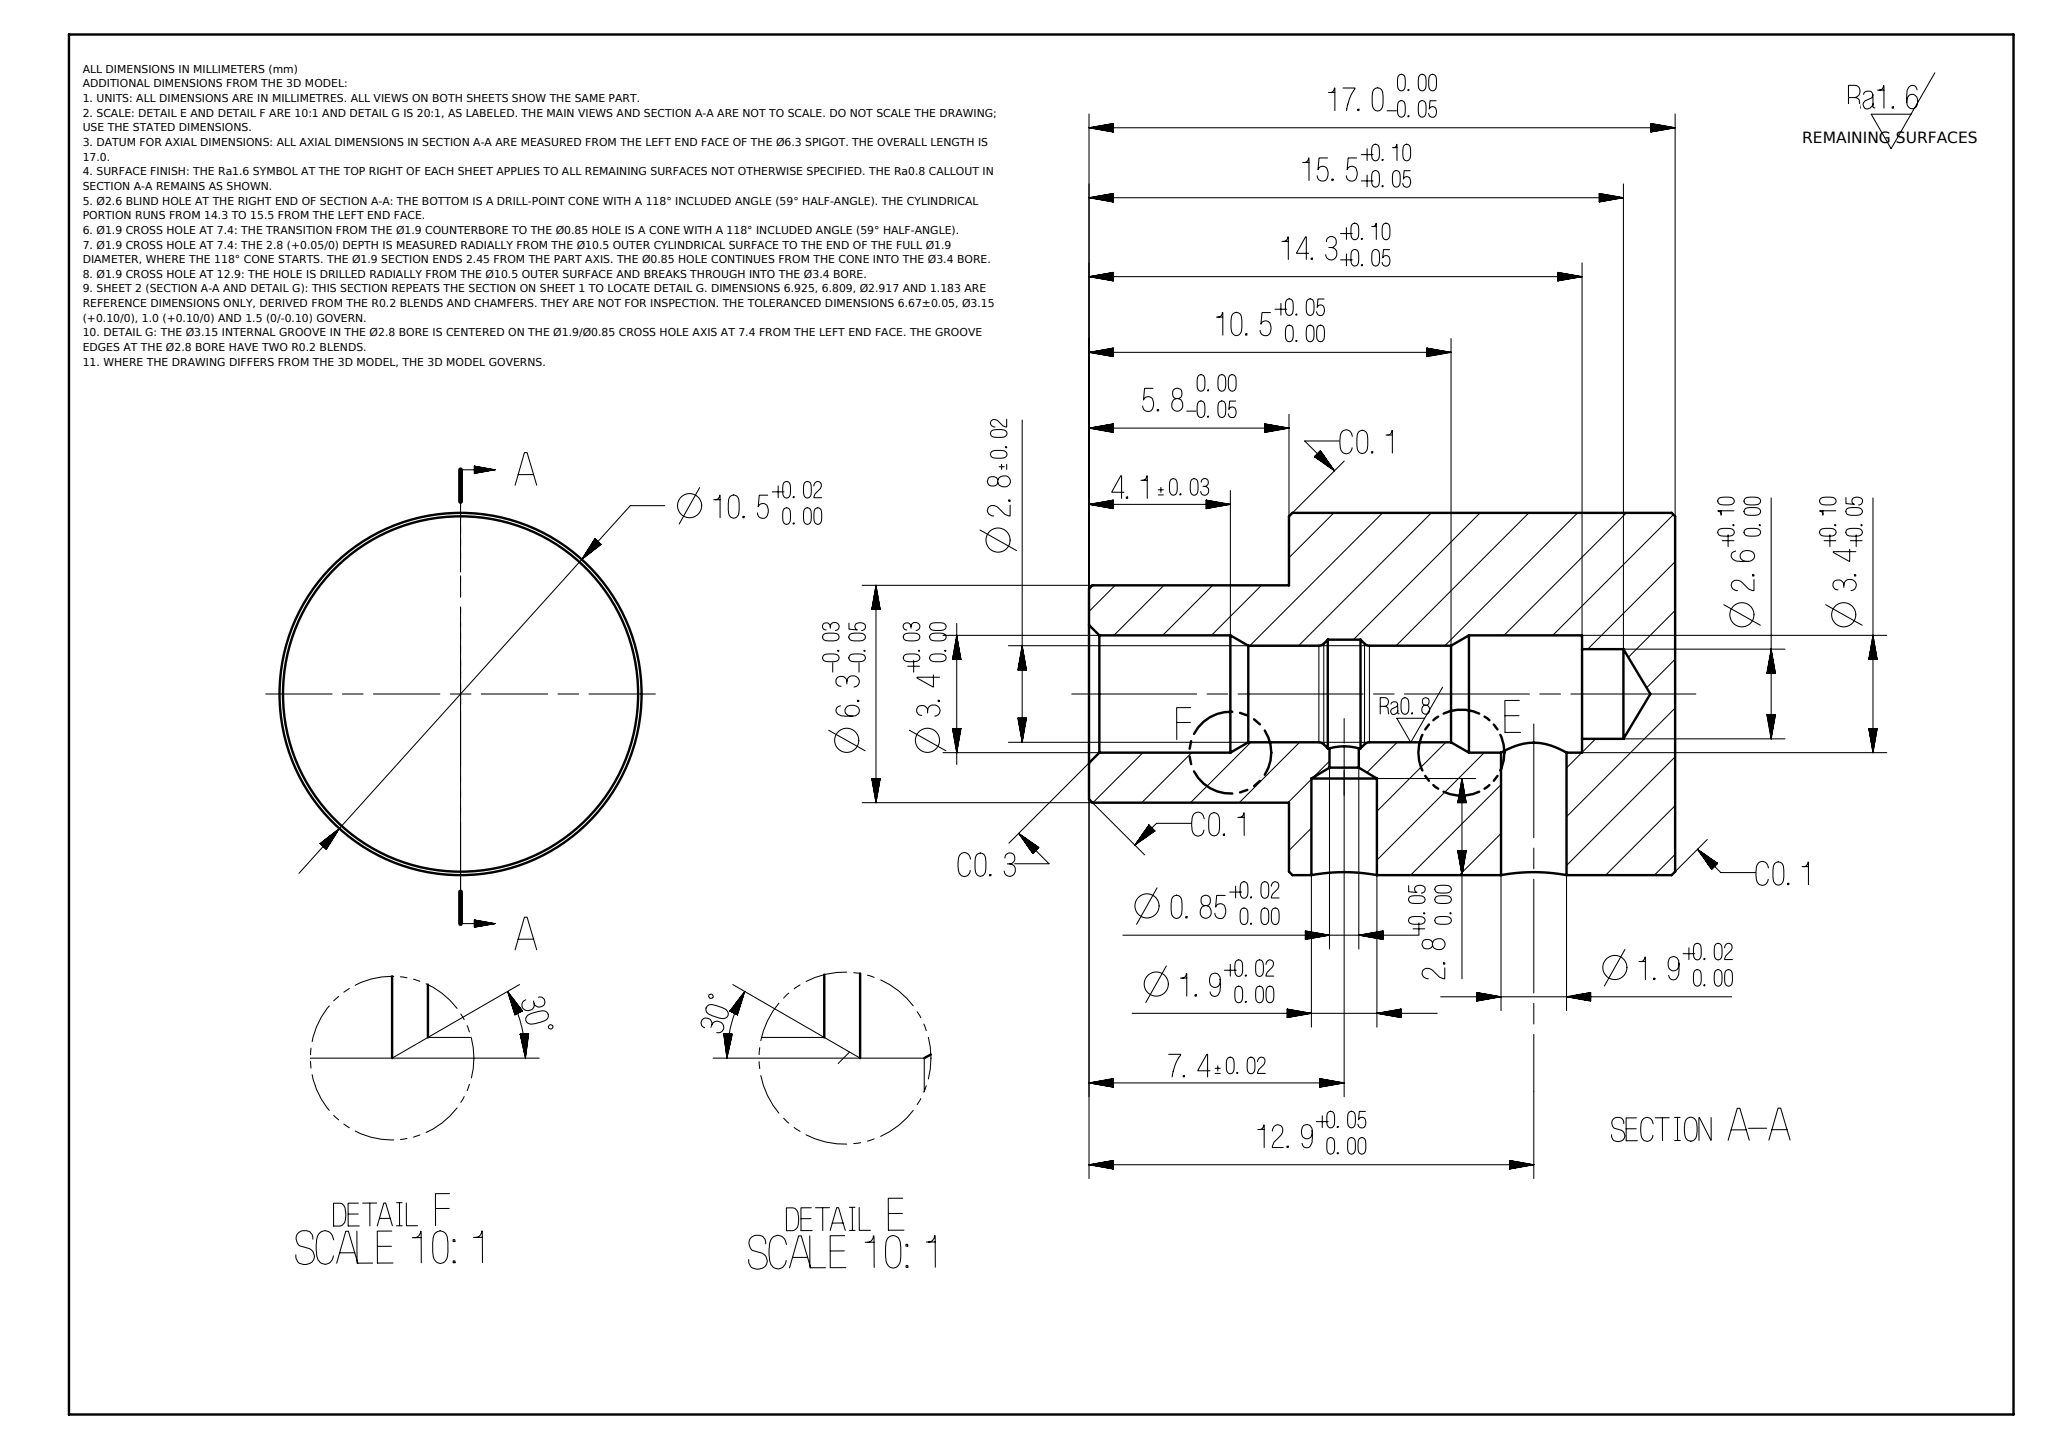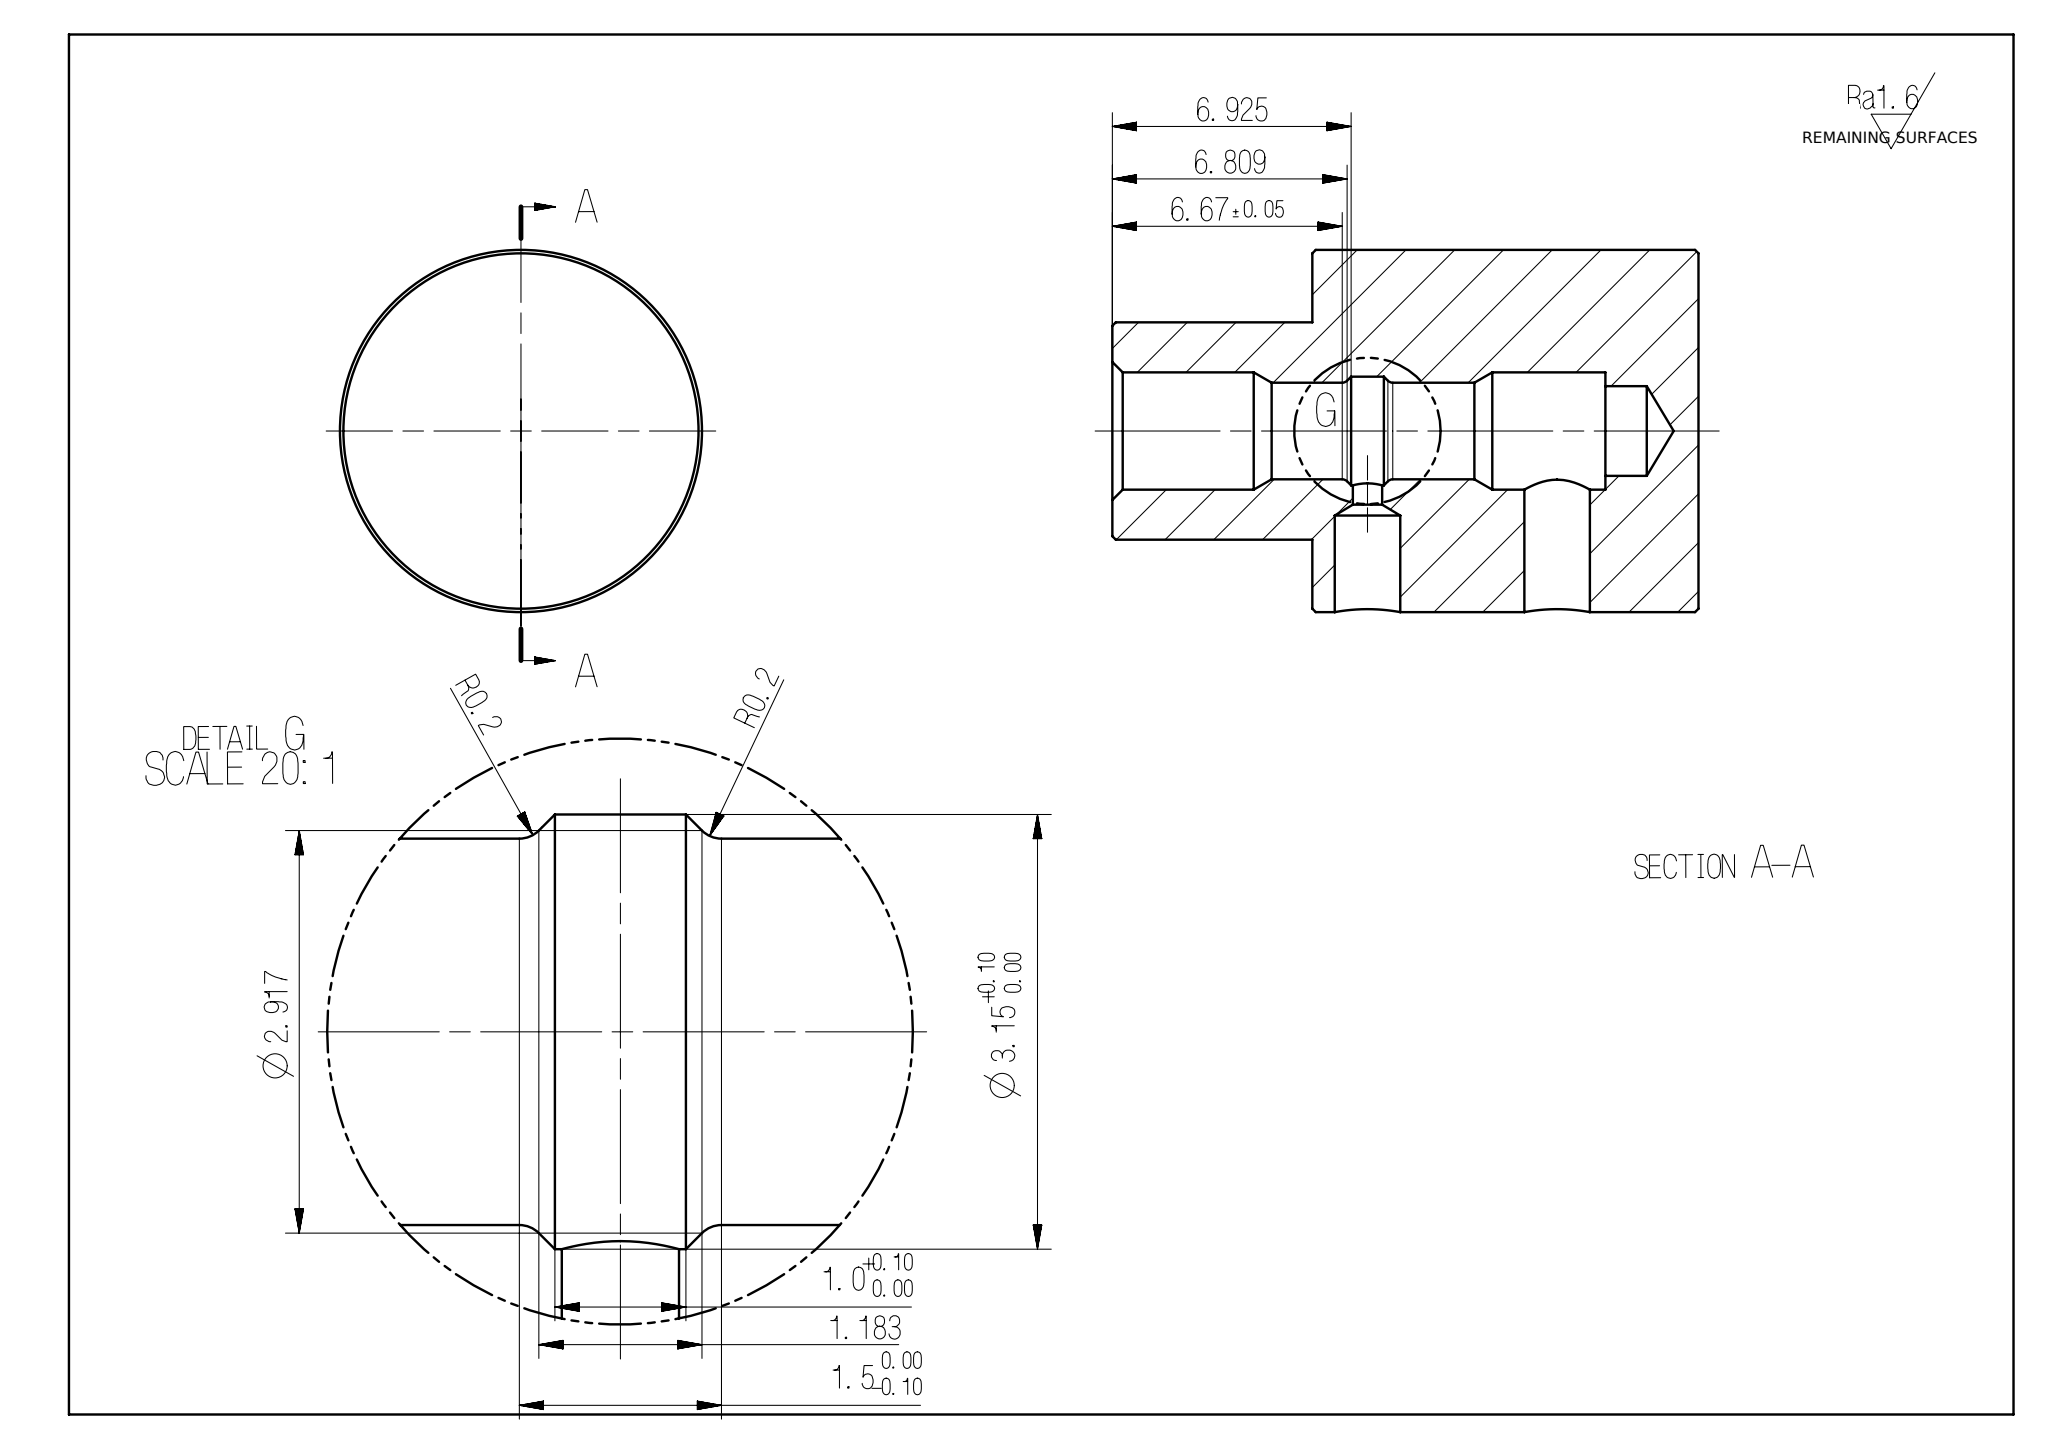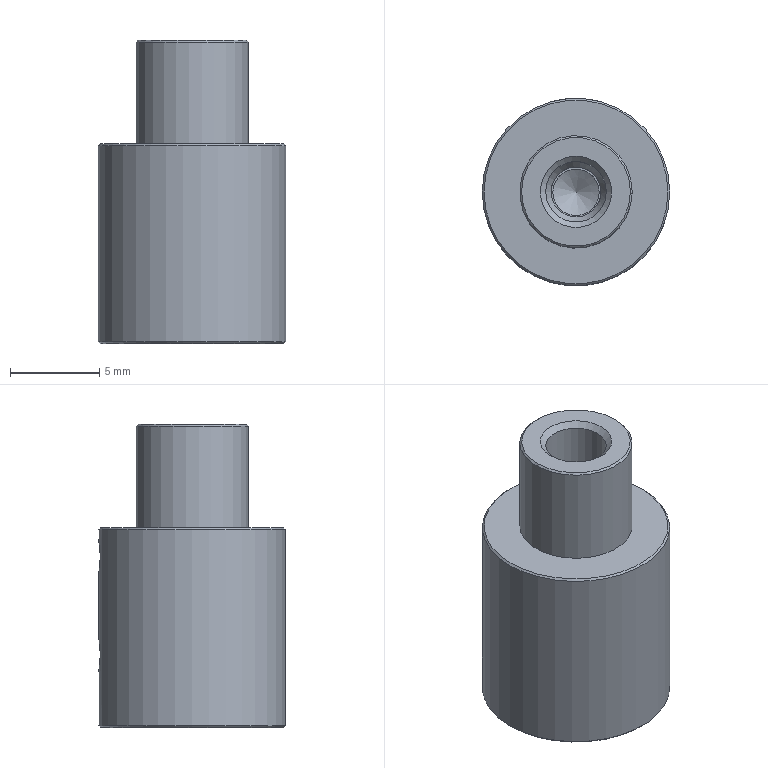Part | NX | mm | 1 solid | 27 faces | box 10.5 x 10.5 x 17 mm | volume 1010 mm3 | cylinder 11 | cone 10 | plane 4 | torus 2 | commonest cylinder face diameters 2.8 x2 3.4 x2 1.9 x2 0.85 x1 10.5 x1 6.3 x1 2.6 x1 3.15 x1
STEP:
#1=CARTESIAN_POINT('',(0.,0.,0.));
#2=DIRECTION('',(0.,0.,1.));
#3=DIRECTION('',(1.,0.,0.));
#4=AXIS2_PLACEMENT_3D('',#1,#2,#3);
#5=(LENGTH_UNIT()NAMED_UNIT(*)SI_UNIT(.MILLI.,.METRE.));
#6=UNCERTAINTY_MEASURE_WITH_UNIT(LENGTH_MEASURE(0.0508),#5,'','');
#7=(NAMED_UNIT(*)PLANE_ANGLE_UNIT()SI_UNIT($,.RADIAN.));
#8=PLANE_ANGLE_MEASURE_WITH_UNIT(PLANE_ANGLE_MEASURE(0.01745),#7);
#9=DIMENSIONAL_EXPONENTS(0.,0.,0.,0.,0.,0.,0.);
#10=(CONVERSION_BASED_UNIT('',#8)NAMED_UNIT(#9)PLANE_ANGLE_UNIT());
#11=(NAMED_UNIT(*)SI_UNIT($,.STERADIAN.)SOLID_ANGLE_UNIT());
#12=(GEOMETRIC_REPRESENTATION_CONTEXT(3)GLOBAL_UNCERTAINTY_ASSIGNED_CONTEXT((#6))GLOBAL_UNIT_ASSIGNED_CONTEXT((#5,#10,#11))REPRESENTATION_CONTEXT('',''));
#13=SHAPE_REPRESENTATION('',(#4),#12);
#14=CARTESIAN_POINT('',(0.,-1.4,10.333));
#15=VERTEX_POINT('',#14);
#16=CARTESIAN_POINT('',(0.,0.,10.333));
#17=DIRECTION('',(0.,-0.,-1.));
#18=DIRECTION('',(0.,-1.,0.));
#19=AXIS2_PLACEMENT_3D('',#16,#17,#18);
#20=CIRCLE('',#19,1.4);
#21=EDGE_CURVE('',#15,#15,#20,.T.);
#22=ORIENTED_EDGE('',*,*,#21,.T.);
#23=EDGE_LOOP('',(#22));
#24=FACE_BOUND('',#23,.T.);
#25=CARTESIAN_POINT('',(-1.4,0.,12.38));
#26=VERTEX_POINT('',#25);
#27=CARTESIAN_POINT('',(0.,0.,12.38));
#28=DIRECTION('',(0.,0.,1.));
#29=DIRECTION('',(-1.,0.,0.));
#30=AXIS2_PLACEMENT_3D('',#27,#28,#29);
#31=CIRCLE('',#30,1.4);
#32=EDGE_CURVE('',#26,#26,#31,.T.);
#33=ORIENTED_EDGE('',*,*,#32,.T.);
#34=EDGE_LOOP('',(#33));
#35=FACE_BOUND('',#34,.T.);
#36=CARTESIAN_POINT('',(0.,0.,6.2));
#37=DIRECTION('',(0.,0.,1.));
#38=DIRECTION('',(1.,0.,0.));
#39=AXIS2_PLACEMENT_3D('',#36,#37,#38);
#40=CYLINDRICAL_SURFACE('',#39,1.4);
#41=ADVANCED_FACE('',(#24,#35),#40,.F.);
#42=CARTESIAN_POINT('',(0.,-1.4,8.867));
#43=VERTEX_POINT('',#42);
#44=CARTESIAN_POINT('',(0.,0.,8.867));
#45=DIRECTION('',(0.,0.,1.));
#46=DIRECTION('',(0.,-1.,0.));
#47=AXIS2_PLACEMENT_3D('',#44,#45,#46);
#48=CIRCLE('',#47,1.4);
#49=EDGE_CURVE('',#43,#43,#48,.T.);
#50=ORIENTED_EDGE('',*,*,#49,.T.);
#51=EDGE_LOOP('',(#50));
#52=FACE_BOUND('',#51,.T.);
#53=CARTESIAN_POINT('',(0.,-1.4,6.5));
#54=VERTEX_POINT('',#53);
#55=CARTESIAN_POINT('',(0.,-0.,6.5));
#56=DIRECTION('',(0.,0.,1.));
#57=DIRECTION('',(0.,-1.,0.));
#58=AXIS2_PLACEMENT_3D('',#55,#56,#57);
#59=CIRCLE('',#58,1.4);
#60=EDGE_CURVE('',#54,#54,#59,.T.);
#61=ORIENTED_EDGE('',*,*,#60,.F.);
#62=EDGE_LOOP('',(#61));
#63=FACE_BOUND('',#62,.T.);
#64=CARTESIAN_POINT('',(0.,0.,6.2));
#65=DIRECTION('',(0.,0.,1.));
#66=DIRECTION('',(1.,0.,0.));
#67=AXIS2_PLACEMENT_3D('',#64,#65,#66);
#68=CYLINDRICAL_SURFACE('',#67,1.4);
#69=ADVANCED_FACE('',(#52,#63),#68,.F.);
#70=CARTESIAN_POINT('',(0.,2.135,10.025));
#71=VERTEX_POINT('',#70);
#72=CARTESIAN_POINT('',(0.,2.135,9.6));
#73=DIRECTION('',(0.,1.,0.));
#74=DIRECTION('',(0.,0.,1.));
#75=AXIS2_PLACEMENT_3D('',#72,#73,#74);
#76=CIRCLE('',#75,0.425);
#77=EDGE_CURVE('',#71,#71,#76,.T.);
#78=ORIENTED_EDGE('',*,*,#77,.T.);
#79=EDGE_LOOP('',(#78));
#80=FACE_BOUND('',#79,.T.);
#81=CARTESIAN_POINT('',(0.425,1.517,9.6));
#82=VERTEX_POINT('',#81);
#83=CARTESIAN_POINT('',(0.425,1.517,9.6));
#84=CARTESIAN_POINT('',(0.425,1.517,9.553));
#85=CARTESIAN_POINT('',(0.4171,1.519,9.506));
#86=CARTESIAN_POINT('',(0.4021,1.523,9.462));
#87=CARTESIAN_POINT('',(0.387,1.527,9.418));
#88=CARTESIAN_POINT('',(0.3645,1.533,9.377));
#89=CARTESIAN_POINT('',(0.3363,1.539,9.34));
#90=CARTESIAN_POINT('',(0.3074,1.545,9.303));
#91=CARTESIAN_POINT('',(0.2718,1.552,9.27));
#92=CARTESIAN_POINT('',(0.2322,1.558,9.244));
#93=CARTESIAN_POINT('',(0.192,1.564,9.218));
#94=CARTESIAN_POINT('',(0.1465,1.569,9.198));
#95=CARTESIAN_POINT('',(0.09951,1.572,9.187));
#96=CARTESIAN_POINT('',(0.05365,1.575,9.176));
#97=CARTESIAN_POINT('',(0.005111,1.576,9.172));
#98=CARTESIAN_POINT('',(-0.0419,1.574,9.177));
#99=CARTESIAN_POINT('',(-0.0877,1.573,9.182));
#100=CARTESIAN_POINT('',(-0.1333,1.57,9.194));
#101=CARTESIAN_POINT('',(-0.175,1.565,9.213));
#102=CARTESIAN_POINT('',(-0.2172,1.561,9.232));
#103=CARTESIAN_POINT('',(-0.2566,1.554,9.258));
#104=CARTESIAN_POINT('',(-0.2903,1.548,9.29));
#105=CARTESIAN_POINT('',(-0.325,1.542,9.322));
#106=CARTESIAN_POINT('',(-0.3546,1.535,9.361));
#107=CARTESIAN_POINT('',(-0.3767,1.529,9.403));
#108=CARTESIAN_POINT('',(-0.3989,1.524,9.446));
#109=CARTESIAN_POINT('',(-0.4141,1.52,9.493));
#110=CARTESIAN_POINT('',(-0.4208,1.518,9.541));
#111=CARTESIAN_POINT('',(-0.4274,1.516,9.587));
#112=CARTESIAN_POINT('',(-0.4261,1.516,9.635));
#113=CARTESIAN_POINT('',(-0.4172,1.519,9.681));
#114=CARTESIAN_POINT('',(-0.4085,1.521,9.726));
#115=CARTESIAN_POINT('',(-0.3922,1.526,9.77));
#116=CARTESIAN_POINT('',(-0.3697,1.531,9.81));
#117=CARTESIAN_POINT('',(-0.3468,1.537,9.85));
#118=CARTESIAN_POINT('',(-0.3167,1.543,9.887));
#119=CARTESIAN_POINT('',(-0.2819,1.55,9.918));
#120=CARTESIAN_POINT('',(-0.2461,1.556,9.95));
#121=CARTESIAN_POINT('',(-0.2043,1.562,9.976));
#122=CARTESIAN_POINT('',(-0.1597,1.567,9.994));
#123=CARTESIAN_POINT('',(-0.1155,1.571,10.012));
#124=CARTESIAN_POINT('',(-0.06734,1.574,10.022));
#125=CARTESIAN_POINT('',(-0.01948,1.575,10.025));
#126=CARTESIAN_POINT('',(0.02689,1.575,10.027));
#127=CARTESIAN_POINT('',(0.07428,1.574,10.021));
#128=CARTESIAN_POINT('',(0.1187,1.571,10.008));
#129=CARTESIAN_POINT('',(0.1629,1.567,9.995));
#130=CARTESIAN_POINT('',(0.2053,1.562,9.975));
#131=CARTESIAN_POINT('',(0.2428,1.556,9.949));
#132=CARTESIAN_POINT('',(0.2814,1.55,9.922));
#133=CARTESIAN_POINT('',(0.3158,1.543,9.888));
#134=CARTESIAN_POINT('',(0.3435,1.537,9.85));
#135=CARTESIAN_POINT('',(0.3717,1.531,9.812));
#136=CARTESIAN_POINT('',(0.3937,1.525,9.767));
#137=CARTESIAN_POINT('',(0.4074,1.521,9.721));
#138=CARTESIAN_POINT('',(0.419,1.518,9.682));
#139=CARTESIAN_POINT('',(0.425,1.517,9.641));
#140=CARTESIAN_POINT('',(0.425,1.517,9.6));
#141=B_SPLINE_CURVE_WITH_KNOTS('',3,(#83,#84,#85,#86,#87,#88,#89,#90,#91,#92,#93,#94,#95,#96,#97,#98,#99,#100,#101,#102,#103,#104,#105,#106,#107,#108,#109,#110,#111,#112,#113,#114,#115,#116,#117,#118,#119,#120,#121,#122,#123,#124,#125,#126,#127,#128,#129,#130,#131,#132,#133,#134,#135,#136,#137,#138,#139,#140),.UNSPECIFIED.,.T.,.F.,(1,3,3,3,3,3,3,3,3,3,3,3,3,3,3,3,3,3,3,3,3,1),(-0.04563,0.,0.05236,0.1046,0.1582,0.2126,0.2657,0.3174,0.3697,0.4236,0.4779,0.5305,0.582,0.6347,0.689,0.7428,0.795,0.8468,0.8999,0.9544,1.,1.052),.UNSPECIFIED.);
#142=EDGE_CURVE('',#82,#82,#141,.T.);
#143=ORIENTED_EDGE('',*,*,#142,.F.);
#144=EDGE_LOOP('',(#143));
#145=FACE_BOUND('',#144,.T.);
#146=CARTESIAN_POINT('',(0.,5.25,9.6));
#147=DIRECTION('',(-0.,-1.,0.));
#148=DIRECTION('',(1.,-0.,0.));
#149=AXIS2_PLACEMENT_3D('',#146,#147,#148);
#150=CYLINDRICAL_SURFACE('',#149,0.425);
#151=ADVANCED_FACE('',(#80,#145),#150,.F.);
#152=CARTESIAN_POINT('',(2.,0.,17.));
#153=VERTEX_POINT('',#152);
#154=CARTESIAN_POINT('',(0.,0.,17.));
#155=DIRECTION('',(0.,0.,-1.));
#156=DIRECTION('',(1.,0.,0.));
#157=AXIS2_PLACEMENT_3D('',#154,#155,#156);
#158=CIRCLE('',#157,2.);
#159=EDGE_CURVE('',#153,#153,#158,.T.);
#160=ORIENTED_EDGE('',*,*,#159,.T.);
#161=EDGE_LOOP('',(#160));
#162=FACE_BOUND('',#161,.T.);
#163=CARTESIAN_POINT('',(3.05,0.,17.));
#164=VERTEX_POINT('',#163);
#165=CARTESIAN_POINT('',(0.,0.,17.));
#166=DIRECTION('',(0.,0.,1.));
#167=DIRECTION('',(1.,0.,0.));
#168=AXIS2_PLACEMENT_3D('',#165,#166,#167);
#169=CIRCLE('',#168,3.05);
#170=EDGE_CURVE('',#164,#164,#169,.T.);
#171=ORIENTED_EDGE('',*,*,#170,.T.);
#172=EDGE_LOOP('',(#171));
#173=FACE_BOUND('',#172,.T.);
#174=CARTESIAN_POINT('',(0.,0.,17.));
#175=DIRECTION('',(0.,0.,1.));
#176=DIRECTION('',(1.,0.,0.));
#177=AXIS2_PLACEMENT_3D('',#174,#175,#176);
#178=PLANE('',#177);
#179=ADVANCED_FACE('',(#162,#173),#178,.T.);
#180=CARTESIAN_POINT('',(-5.15,0.,0.));
#181=VERTEX_POINT('',#180);
#182=CARTESIAN_POINT('',(0.,0.,0.));
#183=DIRECTION('',(0.,0.,-1.));
#184=DIRECTION('',(-1.,0.,0.));
#185=AXIS2_PLACEMENT_3D('',#182,#183,#184);
#186=CIRCLE('',#185,5.15);
#187=EDGE_CURVE('',#181,#181,#186,.T.);
#188=ORIENTED_EDGE('',*,*,#187,.T.);
#189=EDGE_LOOP('',(#188));
#190=FACE_OUTER_BOUND('',#189,.T.);
#191=CARTESIAN_POINT('',(0.,0.,0.));
#192=DIRECTION('',(0.,0.,-1.));
#193=DIRECTION('',(-1.,0.,0.));
#194=AXIS2_PLACEMENT_3D('',#191,#192,#193);
#195=PLANE('',#194);
#196=ADVANCED_FACE('',(#190),#195,.T.);
#197=CARTESIAN_POINT('',(0.,5.25,8.65));
#198=VERTEX_POINT('',#197);
#199=CARTESIAN_POINT('',(0.,5.25,8.65));
#200=CARTESIAN_POINT('',(-0.1054,5.25,8.65));
#201=CARTESIAN_POINT('',(-0.2122,5.247,8.668));
#202=CARTESIAN_POINT('',(-0.3116,5.241,8.703));
#203=CARTESIAN_POINT('',(-0.4109,5.235,8.737));
#204=CARTESIAN_POINT('',(-0.5056,5.226,8.789));
#205=CARTESIAN_POINT('',(-0.588,5.217,8.854));
#206=CARTESIAN_POINT('',(-0.6712,5.208,8.919));
#207=CARTESIAN_POINT('',(-0.7443,5.197,9.));
#208=CARTESIAN_POINT('',(-0.8012,5.189,9.09));
#209=CARTESIAN_POINT('',(-0.8586,5.18,9.18));
#210=CARTESIAN_POINT('',(-0.9012,5.172,9.281));
#211=CARTESIAN_POINT('',(-0.9254,5.168,9.385));
#212=CARTESIAN_POINT('',(-0.9494,5.164,9.488));
#213=CARTESIAN_POINT('',(-0.9559,5.162,9.597));
#214=CARTESIAN_POINT('',(-0.9444,5.164,9.703));
#215=CARTESIAN_POINT('',(-0.9331,5.166,9.807));
#216=CARTESIAN_POINT('',(-0.904,5.172,9.91));
#217=CARTESIAN_POINT('',(-0.8595,5.179,10.005));
#218=CARTESIAN_POINT('',(-0.8148,5.187,10.1));
#219=CARTESIAN_POINT('',(-0.7533,5.196,10.188));
#220=CARTESIAN_POINT('',(-0.6801,5.206,10.263));
#221=CARTESIAN_POINT('',(-0.6058,5.215,10.339));
#222=CARTESIAN_POINT('',(-0.5173,5.225,10.404));
#223=CARTESIAN_POINT('',(-0.4219,5.233,10.451));
#224=CARTESIAN_POINT('',(-0.3263,5.241,10.499));
#225=CARTESIAN_POINT('',(-0.221,5.246,10.53));
#226=CARTESIAN_POINT('',(-0.1149,5.249,10.543));
#227=CARTESIAN_POINT('',(-0.01021,5.251,10.556));
#228=CARTESIAN_POINT('',(0.09817,5.25,10.551));
#229=CARTESIAN_POINT('',(0.2012,5.246,10.528));
#230=CARTESIAN_POINT('',(0.3034,5.242,10.506));
#231=CARTESIAN_POINT('',(0.4032,5.235,10.467));
#232=CARTESIAN_POINT('',(0.4924,5.227,10.412));
#233=CARTESIAN_POINT('',(0.5826,5.218,10.358));
#234=CARTESIAN_POINT('',(0.6646,5.208,10.287));
#235=CARTESIAN_POINT('',(0.7318,5.199,10.206));
#236=CARTESIAN_POINT('',(0.7998,5.189,10.124));
#237=CARTESIAN_POINT('',(0.8546,5.18,10.029));
#238=CARTESIAN_POINT('',(0.8915,5.174,9.928));
#239=CARTESIAN_POINT('',(0.9283,5.167,9.828));
#240=CARTESIAN_POINT('',(0.9483,5.164,9.721));
#241=CARTESIAN_POINT('',(0.9499,5.163,9.614));
#242=CARTESIAN_POINT('',(0.9514,5.163,9.509));
#243=CARTESIAN_POINT('',(0.9351,5.166,9.402));
#244=CARTESIAN_POINT('',(0.9023,5.172,9.303));
#245=CARTESIAN_POINT('',(0.8695,5.178,9.203));
#246=CARTESIAN_POINT('',(0.8195,5.186,9.108));
#247=CARTESIAN_POINT('',(0.7563,5.195,9.025));
#248=CARTESIAN_POINT('',(0.6922,5.205,8.941));
#249=CARTESIAN_POINT('',(0.6128,5.215,8.866));
#250=CARTESIAN_POINT('',(0.5245,5.224,8.808));
#251=CARTESIAN_POINT('',(0.4355,5.233,8.749));
#252=CARTESIAN_POINT('',(0.3348,5.24,8.705));
#253=CARTESIAN_POINT('',(0.231,5.245,8.679));
#254=CARTESIAN_POINT('',(0.1558,5.248,8.66));
#255=CARTESIAN_POINT('',(0.0776,5.25,8.65));
#256=CARTESIAN_POINT('',(0.,5.25,8.65));
#257=B_SPLINE_CURVE_WITH_KNOTS('',3,(#199,#200,#201,#202,#203,#204,#205,#206,#207,#208,#209,#210,#211,#212,#213,#214,#215,#216,#217,#218,#219,#220,#221,#222,#223,#224,#225,#226,#227,#228,#229,#230,#231,#232,#233,#234,#235,#236,#237,#238,#239,#240,#241,#242,#243,#244,#245,#246,#247,#248,#249,#250,#251,#252,#253,#254,#255,#256),.UNSPECIFIED.,.T.,.F.,(1,3,3,3,3,3,3,3,3,3,3,3,3,3,3,3,3,3,3,3,3,1),(-0.03885,0.,0.05311,0.1062,0.1598,0.2138,0.2673,0.32,0.3731,0.4269,0.4808,0.534,0.5868,0.6401,0.6941,0.7478,0.8007,0.8535,0.9071,0.9611,1.,1.053),.UNSPECIFIED.);
#258=EDGE_CURVE('',#198,#198,#257,.T.);
#259=ORIENTED_EDGE('',*,*,#258,.F.);
#260=EDGE_LOOP('',(#259));
#261=FACE_BOUND('',#260,.T.);
#262=CARTESIAN_POINT('',(-5.25,0.,0.1));
#263=VERTEX_POINT('',#262);
#264=CARTESIAN_POINT('',(0.,0.,0.1));
#265=DIRECTION('',(0.,0.,1.));
#266=DIRECTION('',(-1.,0.,0.));
#267=AXIS2_PLACEMENT_3D('',#264,#265,#266);
#268=CIRCLE('',#267,5.25);
#269=EDGE_CURVE('',#263,#263,#268,.T.);
#270=ORIENTED_EDGE('',*,*,#269,.T.);
#271=EDGE_LOOP('',(#270));
#272=FACE_BOUND('',#271,.T.);
#273=CARTESIAN_POINT('',(5.25,0.,11.1));
#274=VERTEX_POINT('',#273);
#275=CARTESIAN_POINT('',(0.,0.,11.1));
#276=DIRECTION('',(0.,0.,-1.));
#277=DIRECTION('',(1.,0.,0.));
#278=AXIS2_PLACEMENT_3D('',#275,#276,#277);
#279=CIRCLE('',#278,5.25);
#280=EDGE_CURVE('',#274,#274,#279,.T.);
#281=ORIENTED_EDGE('',*,*,#280,.T.);
#282=EDGE_LOOP('',(#281));
#283=FACE_BOUND('',#282,.T.);
#284=CARTESIAN_POINT('',(0.,5.25,5.05));
#285=VERTEX_POINT('',#284);
#286=CARTESIAN_POINT('',(0.,5.25,5.05));
#287=CARTESIAN_POINT('',(0.1054,5.25,5.05));
#288=CARTESIAN_POINT('',(0.2122,5.247,5.032));
#289=CARTESIAN_POINT('',(0.3116,5.241,4.997));
#290=CARTESIAN_POINT('',(0.4109,5.235,4.963));
#291=CARTESIAN_POINT('',(0.5056,5.226,4.911));
#292=CARTESIAN_POINT('',(0.588,5.217,4.846));
#293=CARTESIAN_POINT('',(0.6712,5.208,4.781));
#294=CARTESIAN_POINT('',(0.7443,5.197,4.7));
#295=CARTESIAN_POINT('',(0.8012,5.189,4.61));
#296=CARTESIAN_POINT('',(0.8586,5.18,4.52));
#297=CARTESIAN_POINT('',(0.9012,5.172,4.419));
#298=CARTESIAN_POINT('',(0.9254,5.168,4.315));
#299=CARTESIAN_POINT('',(0.9494,5.164,4.212));
#300=CARTESIAN_POINT('',(0.9559,5.162,4.103));
#301=CARTESIAN_POINT('',(0.9444,5.164,3.997));
#302=CARTESIAN_POINT('',(0.9331,5.166,3.893));
#303=CARTESIAN_POINT('',(0.904,5.172,3.79));
#304=CARTESIAN_POINT('',(0.8595,5.179,3.695));
#305=CARTESIAN_POINT('',(0.8148,5.187,3.6));
#306=CARTESIAN_POINT('',(0.7533,5.196,3.512));
#307=CARTESIAN_POINT('',(0.6801,5.206,3.437));
#308=CARTESIAN_POINT('',(0.6058,5.215,3.361));
#309=CARTESIAN_POINT('',(0.5173,5.225,3.296));
#310=CARTESIAN_POINT('',(0.4219,5.233,3.249));
#311=CARTESIAN_POINT('',(0.3263,5.241,3.201));
#312=CARTESIAN_POINT('',(0.221,5.246,3.17));
#313=CARTESIAN_POINT('',(0.1149,5.249,3.157));
#314=CARTESIAN_POINT('',(0.01021,5.251,3.144));
#315=CARTESIAN_POINT('',(-0.09817,5.25,3.149));
#316=CARTESIAN_POINT('',(-0.2012,5.246,3.172));
#317=CARTESIAN_POINT('',(-0.3034,5.242,3.194));
#318=CARTESIAN_POINT('',(-0.4032,5.235,3.233));
#319=CARTESIAN_POINT('',(-0.4924,5.227,3.288));
#320=CARTESIAN_POINT('',(-0.5826,5.218,3.342));
#321=CARTESIAN_POINT('',(-0.6646,5.208,3.413));
#322=CARTESIAN_POINT('',(-0.7318,5.199,3.494));
#323=CARTESIAN_POINT('',(-0.7998,5.189,3.576));
#324=CARTESIAN_POINT('',(-0.8546,5.18,3.671));
#325=CARTESIAN_POINT('',(-0.8915,5.174,3.772));
#326=CARTESIAN_POINT('',(-0.9283,5.167,3.872));
#327=CARTESIAN_POINT('',(-0.9483,5.164,3.979));
#328=CARTESIAN_POINT('',(-0.9499,5.163,4.086));
#329=CARTESIAN_POINT('',(-0.9514,5.163,4.191));
#330=CARTESIAN_POINT('',(-0.9351,5.166,4.298));
#331=CARTESIAN_POINT('',(-0.9023,5.172,4.397));
#332=CARTESIAN_POINT('',(-0.8695,5.178,4.497));
#333=CARTESIAN_POINT('',(-0.8195,5.186,4.592));
#334=CARTESIAN_POINT('',(-0.7563,5.195,4.675));
#335=CARTESIAN_POINT('',(-0.6922,5.205,4.759));
#336=CARTESIAN_POINT('',(-0.6128,5.215,4.834));
#337=CARTESIAN_POINT('',(-0.5245,5.224,4.892));
#338=CARTESIAN_POINT('',(-0.4355,5.233,4.951));
#339=CARTESIAN_POINT('',(-0.3348,5.24,4.995));
#340=CARTESIAN_POINT('',(-0.231,5.245,5.021));
#341=CARTESIAN_POINT('',(-0.1558,5.248,5.04));
#342=CARTESIAN_POINT('',(-0.0776,5.25,5.05));
#343=CARTESIAN_POINT('',(0.,5.25,5.05));
#344=B_SPLINE_CURVE_WITH_KNOTS('',3,(#286,#287,#288,#289,#290,#291,#292,#293,#294,#295,#296,#297,#298,#299,#300,#301,#302,#303,#304,#305,#306,#307,#308,#309,#310,#311,#312,#313,#314,#315,#316,#317,#318,#319,#320,#321,#322,#323,#324,#325,#326,#327,#328,#329,#330,#331,#332,#333,#334,#335,#336,#337,#338,#339,#340,#341,#342,#343),.UNSPECIFIED.,.T.,.F.,(1,3,3,3,3,3,3,3,3,3,3,3,3,3,3,3,3,3,3,3,3,1),(-0.03885,0.,0.05311,0.1062,0.1598,0.2138,0.2673,0.32,0.3731,0.4269,0.4808,0.534,0.5868,0.6401,0.6941,0.7478,0.8007,0.8535,0.9071,0.9611,1.,1.053),.UNSPECIFIED.);
#345=EDGE_CURVE('',#285,#285,#344,.T.);
#346=ORIENTED_EDGE('',*,*,#345,.F.);
#347=EDGE_LOOP('',(#346));
#348=FACE_BOUND('',#347,.T.);
#349=CARTESIAN_POINT('',(0.,0.,0.));
#350=DIRECTION('',(0.,0.,1.));
#351=DIRECTION('',(1.,0.,0.));
#352=AXIS2_PLACEMENT_3D('',#349,#350,#351);
#353=CYLINDRICAL_SURFACE('',#352,5.25);
#354=ADVANCED_FACE('',(#261,#272,#283,#348),#353,.T.);
#355=CARTESIAN_POINT('',(5.15,0.,11.2));
#356=VERTEX_POINT('',#355);
#357=CARTESIAN_POINT('',(0.,0.,11.2));
#358=DIRECTION('',(0.,0.,1.));
#359=DIRECTION('',(1.,0.,0.));
#360=AXIS2_PLACEMENT_3D('',#357,#358,#359);
#361=CIRCLE('',#360,5.15);
#362=EDGE_CURVE('',#356,#356,#361,.T.);
#363=ORIENTED_EDGE('',*,*,#362,.T.);
#364=EDGE_LOOP('',(#363));
#365=FACE_BOUND('',#364,.T.);
#366=CARTESIAN_POINT('',(3.15,0.,11.2));
#367=VERTEX_POINT('',#366);
#368=CARTESIAN_POINT('',(0.,0.,11.2));
#369=DIRECTION('',(0.,0.,1.));
#370=DIRECTION('',(1.,0.,0.));
#371=AXIS2_PLACEMENT_3D('',#368,#369,#370);
#372=CIRCLE('',#371,3.15);
#373=EDGE_CURVE('',#367,#367,#372,.T.);
#374=ORIENTED_EDGE('',*,*,#373,.F.);
#375=EDGE_LOOP('',(#374));
#376=FACE_BOUND('',#375,.T.);
#377=CARTESIAN_POINT('',(0.,0.,11.2));
#378=DIRECTION('',(0.,0.,1.));
#379=DIRECTION('',(1.,0.,0.));
#380=AXIS2_PLACEMENT_3D('',#377,#378,#379);
#381=PLANE('',#380);
#382=ADVANCED_FACE('',(#365,#376),#381,.T.);
#383=CARTESIAN_POINT('',(3.15,0.,16.9));
#384=VERTEX_POINT('',#383);
#385=CARTESIAN_POINT('',(0.,0.,16.9));
#386=DIRECTION('',(0.,0.,-1.));
#387=DIRECTION('',(1.,0.,0.));
#388=AXIS2_PLACEMENT_3D('',#385,#386,#387);
#389=CIRCLE('',#388,3.15);
#390=EDGE_CURVE('',#384,#384,#389,.T.);
#391=ORIENTED_EDGE('',*,*,#390,.T.);
#392=EDGE_LOOP('',(#391));
#393=FACE_BOUND('',#392,.T.);
#394=ORIENTED_EDGE('',*,*,#373,.T.);
#395=EDGE_LOOP('',(#394));
#396=FACE_BOUND('',#395,.T.);
#397=CARTESIAN_POINT('',(0.,0.,11.2));
#398=DIRECTION('',(0.,0.,1.));
#399=DIRECTION('',(1.,0.,0.));
#400=AXIS2_PLACEMENT_3D('',#397,#398,#399);
#401=CYLINDRICAL_SURFACE('',#400,3.15);
#402=ADVANCED_FACE('',(#393,#396),#401,.T.);
#403=CARTESIAN_POINT('',(1.7,0.,16.7));
#404=VERTEX_POINT('',#403);
#405=CARTESIAN_POINT('',(0.,0.,16.7));
#406=DIRECTION('',(0.,0.,1.));
#407=DIRECTION('',(1.,0.,0.));
#408=AXIS2_PLACEMENT_3D('',#405,#406,#407);
#409=CIRCLE('',#408,1.7);
#410=EDGE_CURVE('',#404,#404,#409,.T.);
#411=ORIENTED_EDGE('',*,*,#410,.T.);
#412=EDGE_LOOP('',(#411));
#413=FACE_BOUND('',#412,.T.);
#414=CARTESIAN_POINT('',(-1.7,0.,12.9));
#415=VERTEX_POINT('',#414);
#416=CARTESIAN_POINT('',(0.,0.,12.9));
#417=DIRECTION('',(0.,0.,-1.));
#418=DIRECTION('',(-1.,0.,0.));
#419=AXIS2_PLACEMENT_3D('',#416,#417,#418);
#420=CIRCLE('',#419,1.7);
#421=EDGE_CURVE('',#415,#415,#420,.T.);
#422=ORIENTED_EDGE('',*,*,#421,.T.);
#423=EDGE_LOOP('',(#422));
#424=FACE_BOUND('',#423,.T.);
#425=CARTESIAN_POINT('',(0.,0.,12.9));
#426=DIRECTION('',(0.,0.,1.));
#427=DIRECTION('',(1.,0.,0.));
#428=AXIS2_PLACEMENT_3D('',#425,#426,#427);
#429=CYLINDRICAL_SURFACE('',#428,1.7);
#430=ADVANCED_FACE('',(#413,#424),#429,.F.);
#431=CARTESIAN_POINT('',(-1.3,0.,1.5));
#432=VERTEX_POINT('',#431);
#433=CARTESIAN_POINT('',(0.,0.,1.5));
#434=DIRECTION('',(0.,0.,-1.));
#435=DIRECTION('',(-1.,0.,0.));
#436=AXIS2_PLACEMENT_3D('',#433,#434,#435);
#437=CIRCLE('',#436,1.3);
#438=EDGE_CURVE('',#432,#432,#437,.T.);
#439=ORIENTED_EDGE('',*,*,#438,.F.);
#440=EDGE_LOOP('',(#439));
#441=FACE_BOUND('',#440,.T.);
#442=CARTESIAN_POINT('',(0.,0.,0.7189));
#443=VERTEX_POINT('',#442);
#444=VERTEX_LOOP('',#443);
#445=FACE_BOUND('',#444,.T.);
#446=CARTESIAN_POINT('',(0.,0.,1.5));
#447=DIRECTION('',(0.,0.,1.));
#448=DIRECTION('',(1.,0.,0.));
#449=AXIS2_PLACEMENT_3D('',#446,#447,#448);
#450=CONICAL_SURFACE('',#449,1.3,59.);
#451=ADVANCED_FACE('',(#441,#445),#450,.F.);
#452=CARTESIAN_POINT('',(-1.3,0.,2.7));
#453=VERTEX_POINT('',#452);
#454=CARTESIAN_POINT('',(0.,0.,2.7));
#455=DIRECTION('',(0.,0.,1.));
#456=DIRECTION('',(-1.,0.,0.));
#457=AXIS2_PLACEMENT_3D('',#454,#455,#456);
#458=CIRCLE('',#457,1.3);
#459=EDGE_CURVE('',#453,#453,#458,.T.);
#460=ORIENTED_EDGE('',*,*,#459,.T.);
#461=EDGE_LOOP('',(#460));
#462=FACE_BOUND('',#461,.T.);
#463=ORIENTED_EDGE('',*,*,#438,.T.);
#464=EDGE_LOOP('',(#463));
#465=FACE_BOUND('',#464,.T.);
#466=CARTESIAN_POINT('',(0.,0.,17.));
#467=DIRECTION('',(0.,0.,-1.));
#468=DIRECTION('',(-1.,0.,0.));
#469=AXIS2_PLACEMENT_3D('',#466,#467,#468);
#470=CYLINDRICAL_SURFACE('',#469,1.3);
#471=ADVANCED_FACE('',(#462,#465),#470,.F.);
#472=CARTESIAN_POINT('',(-1.7,0.,2.7));
#473=VERTEX_POINT('',#472);
#474=CARTESIAN_POINT('',(0.,0.,2.7));
#475=DIRECTION('',(0.,0.,-1.));
#476=DIRECTION('',(-1.,0.,0.));
#477=AXIS2_PLACEMENT_3D('',#474,#475,#476);
#478=CIRCLE('',#477,1.7);
#479=EDGE_CURVE('',#473,#473,#478,.T.);
#480=ORIENTED_EDGE('',*,*,#479,.F.);
#481=EDGE_LOOP('',(#480));
#482=FACE_BOUND('',#481,.T.);
#483=ORIENTED_EDGE('',*,*,#459,.F.);
#484=EDGE_LOOP('',(#483));
#485=FACE_BOUND('',#484,.T.);
#486=CARTESIAN_POINT('',(0.,0.,2.7));
#487=DIRECTION('',(0.,0.,-1.));
#488=DIRECTION('',(-1.,0.,0.));
#489=AXIS2_PLACEMENT_3D('',#486,#487,#488);
#490=PLANE('',#489);
#491=ADVANCED_FACE('',(#482,#485),#490,.F.);
#492=CARTESIAN_POINT('',(0.,1.7,5.98));
#493=VERTEX_POINT('',#492);
#494=CARTESIAN_POINT('',(0.,0.,5.98));
#495=DIRECTION('',(0.,-0.,-1.));
#496=DIRECTION('',(0.,1.,-0.));
#497=AXIS2_PLACEMENT_3D('',#494,#495,#496);
#498=CIRCLE('',#497,1.7);
#499=EDGE_CURVE('',#493,#493,#498,.T.);
#500=ORIENTED_EDGE('',*,*,#499,.F.);
#501=EDGE_LOOP('',(#500));
#502=FACE_BOUND('',#501,.T.);
#503=CARTESIAN_POINT('',(0.95,1.41,4.1));
#504=VERTEX_POINT('',#503);
#505=CARTESIAN_POINT('',(0.95,1.41,4.1));
#506=CARTESIAN_POINT('',(0.95,1.41,4.197));
#507=CARTESIAN_POINT('',(0.9347,1.42,4.295));
#508=CARTESIAN_POINT('',(0.9062,1.438,4.385));
#509=CARTESIAN_POINT('',(0.8778,1.456,4.475));
#510=CARTESIAN_POINT('',(0.8358,1.482,4.561));
#511=CARTESIAN_POINT('',(0.7836,1.509,4.637));
#512=CARTESIAN_POINT('',(0.7259,1.539,4.721));
#513=CARTESIAN_POINT('',(0.6542,1.571,4.796));
#514=CARTESIAN_POINT('',(0.5726,1.601,4.858));
#515=CARTESIAN_POINT('',(0.4838,1.632,4.925));
#516=CARTESIAN_POINT('',(0.3803,1.661,4.978));
#517=CARTESIAN_POINT('',(0.2706,1.678,5.011));
#518=CARTESIAN_POINT('',(0.1705,1.694,5.04));
#519=CARTESIAN_POINT('',(0.06206,1.702,5.054));
#520=CARTESIAN_POINT('',(-0.04352,1.699,5.049));
#521=CARTESIAN_POINT('',(-0.1378,1.697,5.045));
#522=CARTESIAN_POINT('',(-0.2323,1.686,5.026));
#523=CARTESIAN_POINT('',(-0.3198,1.67,4.995));
#524=CARTESIAN_POINT('',(-0.4082,1.653,4.963));
#525=CARTESIAN_POINT('',(-0.4916,1.629,4.918));
#526=CARTESIAN_POINT('',(-0.5654,1.603,4.863));
#527=CARTESIAN_POINT('',(-0.6473,1.574,4.803));
#528=CARTESIAN_POINT('',(-0.7195,1.542,4.729));
#529=CARTESIAN_POINT('',(-0.7778,1.512,4.645));
#530=CARTESIAN_POINT('',(-0.8415,1.479,4.555));
#531=CARTESIAN_POINT('',(-0.8905,1.448,4.45));
#532=CARTESIAN_POINT('',(-0.9193,1.43,4.34));
#533=CARTESIAN_POINT('',(-0.9457,1.413,4.238));
#534=CARTESIAN_POINT('',(-0.9555,1.406,4.128));
#535=CARTESIAN_POINT('',(-0.9469,1.412,4.023));
#536=CARTESIAN_POINT('',(-0.9396,1.417,3.933));
#537=CARTESIAN_POINT('',(-0.9191,1.431,3.844));
#538=CARTESIAN_POINT('',(-0.8878,1.45,3.762));
#539=CARTESIAN_POINT('',(-0.8552,1.47,3.676));
#540=CARTESIAN_POINT('',(-0.8101,1.496,3.596));
#541=CARTESIAN_POINT('',(-0.7557,1.523,3.524));
#542=CARTESIAN_POINT('',(-0.6922,1.554,3.441));
#543=CARTESIAN_POINT('',(-0.6143,1.588,3.368));
#544=CARTESIAN_POINT('',(-0.5265,1.616,3.309));
#545=CARTESIAN_POINT('',(-0.434,1.647,3.248));
#546=CARTESIAN_POINT('',(-0.3272,1.672,3.201));
#547=CARTESIAN_POINT('',(-0.2158,1.686,3.175));
#548=CARTESIAN_POINT('',(-0.1161,1.699,3.152));
#549=CARTESIAN_POINT('',(-0.009569,1.703,3.144));
#550=CARTESIAN_POINT('',(0.09303,1.697,3.155));
#551=CARTESIAN_POINT('',(0.1861,1.692,3.164));
#552=CARTESIAN_POINT('',(0.2784,1.679,3.187));
#553=CARTESIAN_POINT('',(0.3632,1.661,3.222));
#554=CARTESIAN_POINT('',(0.4508,1.642,3.258));
#555=CARTESIAN_POINT('',(0.5326,1.616,3.308));
#556=CARTESIAN_POINT('',(0.6042,1.589,3.367));
#557=CARTESIAN_POINT('',(0.6842,1.559,3.433));
#558=CARTESIAN_POINT('',(0.7537,1.525,3.512));
#559=CARTESIAN_POINT('',(0.8083,1.496,3.601));
#560=CARTESIAN_POINT('',(0.8668,1.464,3.696));
#561=CARTESIAN_POINT('',(0.91,1.436,3.804));
#562=CARTESIAN_POINT('',(0.9322,1.422,3.917));
#563=CARTESIAN_POINT('',(0.9439,1.414,3.977));
#564=CARTESIAN_POINT('',(0.95,1.41,4.038));
#565=CARTESIAN_POINT('',(0.95,1.41,4.1));
#566=B_SPLINE_CURVE_WITH_KNOTS('',3,(#505,#506,#507,#508,#509,#510,#511,#512,#513,#514,#515,#516,#517,#518,#519,#520,#521,#522,#523,#524,#525,#526,#527,#528,#529,#530,#531,#532,#533,#534,#535,#536,#537,#538,#539,#540,#541,#542,#543,#544,#545,#546,#547,#548,#549,#550,#551,#552,#553,#554,#555,#556,#557,#558,#559,#560,#561,#562,#563,#564,#565),.UNSPECIFIED.,.T.,.F.,(1,3,3,3,3,3,3,3,3,3,3,3,3,3,3,3,3,3,3,3,3,3,1),(-0.03004,0.,0.04782,0.09529,0.1478,0.2052,0.2576,0.3041,0.3511,0.4034,0.4607,0.5133,0.5577,0.6038,0.6577,0.7147,0.7658,0.8119,0.8594,0.9127,0.97,1.,1.048),.UNSPECIFIED.);
#567=EDGE_CURVE('',#504,#504,#566,.T.);
#568=ORIENTED_EDGE('',*,*,#567,.F.);
#569=EDGE_LOOP('',(#568));
#570=FACE_BOUND('',#569,.T.);
#571=ORIENTED_EDGE('',*,*,#479,.T.);
#572=EDGE_LOOP('',(#571));
#573=FACE_BOUND('',#572,.T.);
#574=CARTESIAN_POINT('',(0.,0.,2.7));
#575=DIRECTION('',(0.,0.,1.));
#576=DIRECTION('',(1.,0.,0.));
#577=AXIS2_PLACEMENT_3D('',#574,#575,#576);
#578=CYLINDRICAL_SURFACE('',#577,1.7);
#579=ADVANCED_FACE('',(#502,#570,#573),#578,.F.);
#580=ORIENTED_EDGE('',*,*,#345,.T.);
#581=EDGE_LOOP('',(#580));
#582=FACE_BOUND('',#581,.T.);
#583=ORIENTED_EDGE('',*,*,#567,.T.);
#584=EDGE_LOOP('',(#583));
#585=FACE_BOUND('',#584,.T.);
#586=CARTESIAN_POINT('',(0.,5.25,4.1));
#587=DIRECTION('',(-0.,-1.,0.));
#588=DIRECTION('',(1.,-0.,0.));
#589=AXIS2_PLACEMENT_3D('',#586,#587,#588);
#590=CYLINDRICAL_SURFACE('',#589,0.95);
#591=ADVANCED_FACE('',(#582,#585),#590,.F.);
#592=ORIENTED_EDGE('',*,*,#170,.F.);
#593=EDGE_LOOP('',(#592));
#594=FACE_BOUND('',#593,.T.);
#595=ORIENTED_EDGE('',*,*,#390,.F.);
#596=EDGE_LOOP('',(#595));
#597=FACE_BOUND('',#596,.T.);
#598=CARTESIAN_POINT('',(0.,0.,16.9));
#599=DIRECTION('',(0.,0.,-1.));
#600=DIRECTION('',(-1.,0.,0.));
#601=AXIS2_PLACEMENT_3D('',#598,#599,#600);
#602=CONICAL_SURFACE('',#601,3.15,45.);
#603=ADVANCED_FACE('',(#594,#597),#602,.T.);
#604=ORIENTED_EDGE('',*,*,#362,.F.);
#605=EDGE_LOOP('',(#604));
#606=FACE_BOUND('',#605,.T.);
#607=ORIENTED_EDGE('',*,*,#280,.F.);
#608=EDGE_LOOP('',(#607));
#609=FACE_BOUND('',#608,.T.);
#610=CARTESIAN_POINT('',(0.,0.,11.1));
#611=DIRECTION('',(0.,0.,-1.));
#612=DIRECTION('',(-1.,0.,-0.));
#613=AXIS2_PLACEMENT_3D('',#610,#611,#612);
#614=CONICAL_SURFACE('',#613,5.25,45.);
#615=ADVANCED_FACE('',(#606,#609),#614,.T.);
#616=ORIENTED_EDGE('',*,*,#187,.F.);
#617=EDGE_LOOP('',(#616));
#618=FACE_BOUND('',#617,.T.);
#619=ORIENTED_EDGE('',*,*,#269,.F.);
#620=EDGE_LOOP('',(#619));
#621=FACE_BOUND('',#620,.T.);
#622=CARTESIAN_POINT('',(0.,0.,0.1));
#623=DIRECTION('',(0.,0.,1.));
#624=DIRECTION('',(1.,0.,-0.));
#625=AXIS2_PLACEMENT_3D('',#622,#623,#624);
#626=CONICAL_SURFACE('',#625,5.25,45.);
#627=ADVANCED_FACE('',(#618,#621),#626,.T.);
#628=ORIENTED_EDGE('',*,*,#410,.F.);
#629=EDGE_LOOP('',(#628));
#630=FACE_BOUND('',#629,.T.);
#631=ORIENTED_EDGE('',*,*,#159,.F.);
#632=EDGE_LOOP('',(#631));
#633=FACE_BOUND('',#632,.T.);
#634=CARTESIAN_POINT('',(0.,0.,17.));
#635=DIRECTION('',(0.,0.,1.));
#636=DIRECTION('',(1.,0.,-0.));
#637=AXIS2_PLACEMENT_3D('',#634,#635,#636);
#638=CONICAL_SURFACE('',#637,2.,45.);
#639=ADVANCED_FACE('',(#630,#633),#638,.F.);
#640=ORIENTED_EDGE('',*,*,#32,.F.);
#641=EDGE_LOOP('',(#640));
#642=FACE_BOUND('',#641,.T.);
#643=ORIENTED_EDGE('',*,*,#421,.F.);
#644=EDGE_LOOP('',(#643));
#645=FACE_BOUND('',#644,.T.);
#646=CARTESIAN_POINT('',(0.,0.,12.9));
#647=DIRECTION('',(0.,0.,1.));
#648=DIRECTION('',(1.,0.,-0.));
#649=AXIS2_PLACEMENT_3D('',#646,#647,#648);
#650=CONICAL_SURFACE('',#649,1.7,30.);
#651=ADVANCED_FACE('',(#642,#645),#650,.F.);
#652=ORIENTED_EDGE('',*,*,#60,.T.);
#653=EDGE_LOOP('',(#652));
#654=FACE_BOUND('',#653,.T.);
#655=ORIENTED_EDGE('',*,*,#499,.T.);
#656=EDGE_LOOP('',(#655));
#657=FACE_BOUND('',#656,.T.);
#658=CARTESIAN_POINT('',(0.,0.,5.98));
#659=DIRECTION('',(0.,-0.,-1.));
#660=DIRECTION('',(0.,1.,-0.));
#661=AXIS2_PLACEMENT_3D('',#658,#659,#660);
#662=CONICAL_SURFACE('',#661,1.7,30.);
#663=ADVANCED_FACE('',(#654,#657),#662,.F.);
#664=CARTESIAN_POINT('',(0.,2.45,8.65));
#665=VERTEX_POINT('',#664);
#666=CARTESIAN_POINT('',(0.,2.45,9.6));
#667=DIRECTION('',(0.,-1.,0.));
#668=DIRECTION('',(0.,0.,-1.));
#669=AXIS2_PLACEMENT_3D('',#666,#667,#668);
#670=CIRCLE('',#669,0.95);
#671=EDGE_CURVE('',#665,#665,#670,.T.);
#672=ORIENTED_EDGE('',*,*,#671,.F.);
#673=EDGE_LOOP('',(#672));
#674=FACE_BOUND('',#673,.T.);
#675=ORIENTED_EDGE('',*,*,#77,.F.);
#676=EDGE_LOOP('',(#675));
#677=FACE_BOUND('',#676,.T.);
#678=CARTESIAN_POINT('',(0.,2.45,9.6));
#679=DIRECTION('',(0.,1.,0.));
#680=DIRECTION('',(0.,0.,1.));
#681=AXIS2_PLACEMENT_3D('',#678,#679,#680);
#682=CONICAL_SURFACE('',#681,0.95,59.);
#683=ADVANCED_FACE('',(#674,#677),#682,.F.);
#684=ORIENTED_EDGE('',*,*,#258,.T.);
#685=EDGE_LOOP('',(#684));
#686=FACE_BOUND('',#685,.T.);
#687=ORIENTED_EDGE('',*,*,#671,.T.);
#688=EDGE_LOOP('',(#687));
#689=FACE_BOUND('',#688,.T.);
#690=CARTESIAN_POINT('',(0.,5.25,9.6));
#691=DIRECTION('',(0.,-1.,0.));
#692=DIRECTION('',(0.,0.,-1.));
#693=AXIS2_PLACEMENT_3D('',#690,#691,#692);
#694=CYLINDRICAL_SURFACE('',#693,0.95);
#695=ADVANCED_FACE('',(#686,#689),#694,.F.);
#696=CARTESIAN_POINT('',(0.,1.575,10.075));
#697=VERTEX_POINT('',#696);
#698=CARTESIAN_POINT('',(0.,-0.,10.075));
#699=DIRECTION('',(0.,-0.,-1.));
#700=DIRECTION('',(0.,1.,-0.));
#701=AXIS2_PLACEMENT_3D('',#698,#699,#700);
#702=CIRCLE('',#701,1.575);
#703=EDGE_CURVE('',#697,#697,#702,.T.);
#704=ORIENTED_EDGE('',*,*,#703,.F.);
#705=EDGE_LOOP('',(#704));
#706=FACE_BOUND('',#705,.T.);
#707=CARTESIAN_POINT('',(0.,1.575,9.125));
#708=VERTEX_POINT('',#707);
#709=CARTESIAN_POINT('',(0.,-0.,9.125));
#710=DIRECTION('',(0.,-0.,-1.));
#711=DIRECTION('',(0.,1.,-0.));
#712=AXIS2_PLACEMENT_3D('',#709,#710,#711);
#713=CIRCLE('',#712,1.575);
#714=EDGE_CURVE('',#708,#708,#713,.T.);
#715=ORIENTED_EDGE('',*,*,#714,.T.);
#716=EDGE_LOOP('',(#715));
#717=FACE_BOUND('',#716,.T.);
#718=ORIENTED_EDGE('',*,*,#142,.T.);
#719=EDGE_LOOP('',(#718));
#720=FACE_BOUND('',#719,.T.);
#721=CARTESIAN_POINT('',(0.,-0.,8.95));
#722=DIRECTION('',(0.,-0.,-1.));
#723=DIRECTION('',(0.,1.,-0.));
#724=AXIS2_PLACEMENT_3D('',#721,#722,#723);
#725=CYLINDRICAL_SURFACE('',#724,1.575);
#726=ADVANCED_FACE('',(#706,#717,#720),#725,.F.);
#727=CARTESIAN_POINT('',(0.,-1.459,10.191));
#728=VERTEX_POINT('',#727);
#729=CARTESIAN_POINT('',(0.,-0.,10.191));
#730=DIRECTION('',(0.,0.,1.));
#731=DIRECTION('',(0.,-1.,0.));
#732=AXIS2_PLACEMENT_3D('',#729,#730,#731);
#733=CIRCLE('',#732,1.459);
#734=EDGE_CURVE('',#728,#728,#733,.T.);
#735=ORIENTED_EDGE('',*,*,#734,.T.);
#736=EDGE_LOOP('',(#735));
#737=FACE_BOUND('',#736,.T.);
#738=ORIENTED_EDGE('',*,*,#703,.T.);
#739=EDGE_LOOP('',(#738));
#740=FACE_BOUND('',#739,.T.);
#741=CARTESIAN_POINT('',(0.,-0.,10.25));
#742=DIRECTION('',(0.,-0.,-1.));
#743=DIRECTION('',(0.,1.,-0.));
#744=AXIS2_PLACEMENT_3D('',#741,#742,#743);
#745=CONICAL_SURFACE('',#744,1.4,45.);
#746=ADVANCED_FACE('',(#737,#740),#745,.F.);
#747=CARTESIAN_POINT('',(0.,1.459,9.009));
#748=VERTEX_POINT('',#747);
#749=CARTESIAN_POINT('',(0.,-0.,9.009));
#750=DIRECTION('',(0.,-0.,-1.));
#751=DIRECTION('',(0.,1.,-0.));
#752=AXIS2_PLACEMENT_3D('',#749,#750,#751);
#753=CIRCLE('',#752,1.459);
#754=EDGE_CURVE('',#748,#748,#753,.T.);
#755=ORIENTED_EDGE('',*,*,#754,.T.);
#756=EDGE_LOOP('',(#755));
#757=FACE_BOUND('',#756,.T.);
#758=ORIENTED_EDGE('',*,*,#714,.F.);
#759=EDGE_LOOP('',(#758));
#760=FACE_BOUND('',#759,.T.);
#761=CARTESIAN_POINT('',(0.,-0.,9.125));
#762=DIRECTION('',(0.,0.,1.));
#763=DIRECTION('',(0.,-1.,0.));
#764=AXIS2_PLACEMENT_3D('',#761,#762,#763);
#765=CONICAL_SURFACE('',#764,1.575,45.);
#766=ADVANCED_FACE('',(#757,#760),#765,.F.);
#767=ORIENTED_EDGE('',*,*,#49,.F.);
#768=EDGE_LOOP('',(#767));
#769=FACE_BOUND('',#768,.T.);
#770=ORIENTED_EDGE('',*,*,#754,.F.);
#771=EDGE_LOOP('',(#770));
#772=FACE_BOUND('',#771,.T.);
#773=CARTESIAN_POINT('',(0.,-0.,8.867));
#774=DIRECTION('',(0.,0.,1.));
#775=DIRECTION('',(0.,-1.,0.));
#776=AXIS2_PLACEMENT_3D('',#773,#774,#775);
#777=TOROIDAL_SURFACE('',#776,1.6,0.2);
#778=ADVANCED_FACE('',(#769,#772),#777,.T.);
#779=ORIENTED_EDGE('',*,*,#734,.F.);
#780=EDGE_LOOP('',(#779));
#781=FACE_BOUND('',#780,.T.);
#782=ORIENTED_EDGE('',*,*,#21,.F.);
#783=EDGE_LOOP('',(#782));
#784=FACE_BOUND('',#783,.T.);
#785=CARTESIAN_POINT('',(0.,-0.,10.333));
#786=DIRECTION('',(0.,0.,1.));
#787=DIRECTION('',(0.,-1.,0.));
#788=AXIS2_PLACEMENT_3D('',#785,#786,#787);
#789=TOROIDAL_SURFACE('',#788,1.6,0.2);
#790=ADVANCED_FACE('',(#781,#784),#789,.T.);
#791=CLOSED_SHELL('',(#41,#69,#151,#179,#196,#354,#382,#402,#430,#451,#471,#491,#579,#591,#603,#615,#627,#639,#651,#663,#683,#695,#726,#746,#766,#778,#790));
#792=MANIFOLD_SOLID_BREP('',#791);
#793=ADVANCED_BREP_SHAPE_REPRESENTATION('',(#792),#12);
#794=SHAPE_REPRESENTATION_RELATIONSHIP('','',#13,#793);
#795=PRESENTATION_LAYER_ASSIGNMENT('','',(#792));
#796=COLOUR_RGB('',0.5961,0.6667,0.6863);
#797=FILL_AREA_STYLE_COLOUR('',#796);
#798=FILL_AREA_STYLE('',(#797));
#799=SURFACE_STYLE_FILL_AREA(#798);
#800=SURFACE_SIDE_STYLE('',(#799));
#801=SURFACE_STYLE_USAGE(.BOTH.,#800);
#802=PRESENTATION_STYLE_ASSIGNMENT((#801));
#803=STYLED_ITEM('',(#802),#792);
#804=MECHANICAL_DESIGN_GEOMETRIC_PRESENTATION_REPRESENTATION('',(#803),#12);